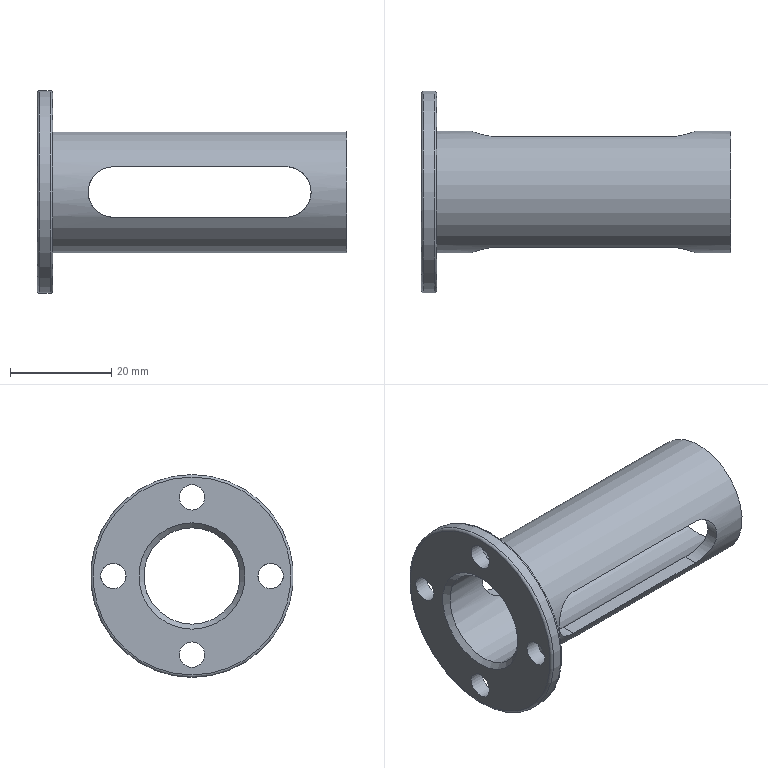Component | NX | CONNECTING_ROD_SUPPORT | 1 solid | 21 faces | volume 10259 mm3 | cylinder 11 | plane 7 | torus 2 | cone 1 | commonest cylinder face diameters 10 x4 5 x4 40 x1 24 x1 19 x1